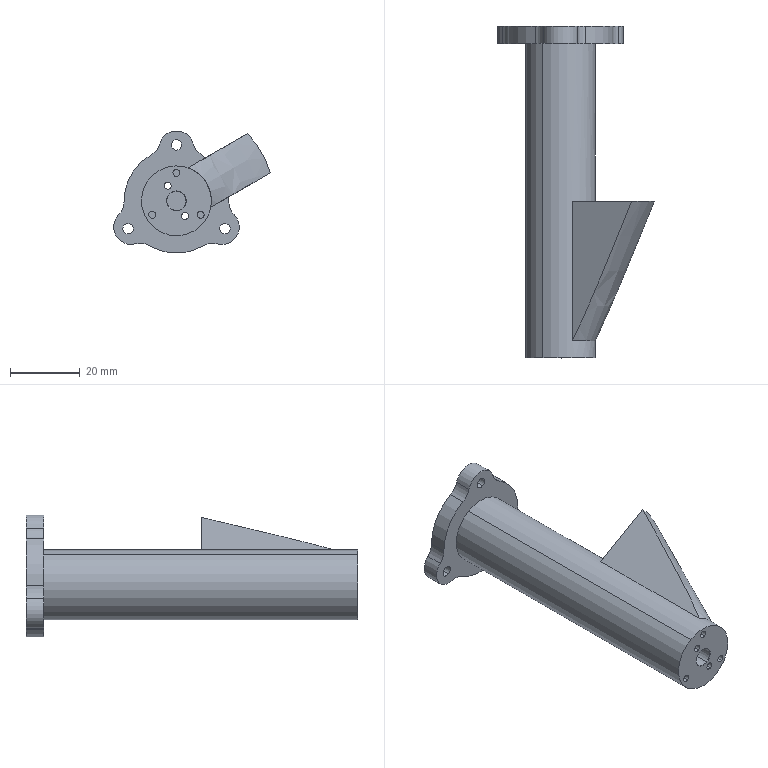Component | SolidWorks | Nozzle1-1 | 1 solid | 58 faces | box 44.86 x 95 x 35 mm | volume 30330 mm3 | cylinder 41 | plane 12 | cone 5 | commonest cylinder face diameters 10 x11 2 x10 3 x8 30 x4 5 x2 13 x2 20 x2 5.5 x2
build123d program:
from build123d import *

# Parameters (mm, degrees)
CUT_EXTRUDE1_REACH       = 101.121
SKETCH4_R                = 1
CUT_EXTRUDE3_START       = -5
SKETCH5_R                = 20
CUT_EXTRUDE3_DEPTH       = 5
FILLET1_R                = 5
SKETCH6_R                = 2.75
CUT_EXTRUDE4_DEPTH       = 20
CUT_EXTRUDE5_REACH       = 100.735
SKETCH7_R                = 1.5
SKETCH12_R               = 1
CUT_EXTRUDE8_DEPTH       = 5
CHAMFER2_SIZE            = 0.08
BOSS_EXTRUDE1_REACH      = 74.782
BOSS_EXTRUDE1_END_RADIUS = 10
SKETCH16_W               = 40
SKETCH16_H               = 13
CUT_EXTRUDE7_REACH       = 77.197
CUT_EXTRUDE7_END_RADIUS  = 2.75
SKETCH11_R               = 1.5
SKETCH25_R               = 2.5
CUT_EXTRUDE10_DEPTH      = 20


with BuildPart() as part:
    # Sketch2 → Revolve1 (revolve)
    with BuildSketch(Plane.XY, mode=Mode.PRIVATE) as revolve1_sk:
        Polygon((-49.735, 0), (45.265, 0), (45.265, 10), (-44.735, 10), (-44.735, 20), (-49.735, 20), align=None)
    revolve(revolve1_sk.sketch.rotate(Axis((-49.735, 0, 0), (1, 0, 0)), 90), axis=Axis((-49.735, 0, 0), (1, 0, 0)))

    # Sketch3 → Cut-Revolve1 (revolve, cut)
    with BuildSketch(Plane(origin=(0, 0, 0), x_dir=(1, 0, 0), z_dir=(0, 1, 0)), mode=Mode.PRIVATE) as cut_revolve1_sk:
        Polygon((-44.735, 6.5), (-49.735, 10), (-49.735, 0), (-9.735, 0), (-9.735, 6.5), align=None)
    revolve(cut_revolve1_sk.sketch.rotate(Axis((-53.807, 0, 0), (1, 0, 0)), 180), axis=Axis((-53.807, 0, 0), (1, 0, 0)), mode=Mode.SUBTRACT)

    # Sketch4 → Cut-Extrude1 (cut, up to next)
    with BuildSketch(Plane(origin=(45.265, 0, 0), x_dir=(0, 0, -1), z_dir=(1, 0, 0)), mode=Mode.PRIVATE) as cut_extrude1_sk1:
        with Locations((5, 0)):
            Circle(SKETCH4_R)
    cut_extrude1_tool1 = extrude(cut_extrude1_sk1.sketch, amount=-CUT_EXTRUDE1_REACH, mode=Mode.PRIVATE) & part.part
    # Sketch4 → Cut-Extrude1 (cut, up to next)
    with BuildSketch(Plane(origin=(45.265, 0, 0), x_dir=(0, 0, -1), z_dir=(1, 0, 0)), mode=Mode.PRIVATE) as cut_extrude1_sk2:
        with Locations(Location((-5, 0, 0), (0, 0, 180))):
            Circle(SKETCH4_R)
    cut_extrude1_tool2 = extrude(cut_extrude1_sk2.sketch, amount=-CUT_EXTRUDE1_REACH, mode=Mode.PRIVATE) & part.part
    add(cut_extrude1_tool1.solids().sort_by_distance((45.265, 0, -5))[0], mode=Mode.SUBTRACT)
    add(cut_extrude1_tool2.solids().sort_by_distance((45.265, 0, 5))[0], mode=Mode.SUBTRACT)

    # Sketch5 → Cut-Extrude3 (cut)
    with BuildSketch(Plane.ZY.offset(49.735).offset(CUT_EXTRUDE3_START)):
        Circle(SKETCH5_R)
        with BuildLine():
            ThreePointArc((4.93, 14.167), (0, 20), (-4.93, 14.167))
            ThreePointArc((-4.93, 14.167), (-12.99, 7.5), (-14.734, -2.814))
            ThreePointArc((-14.734, -2.814), (-17.321, -10), (-9.804, -11.353))
            ThreePointArc((-9.804, -11.353), (0, -15), (9.804, -11.353))
            ThreePointArc((9.804, -11.353), (17.321, -10), (14.734, -2.814))
            ThreePointArc((14.734, -2.814), (12.99, 7.5), (4.93, 14.167))
        make_face(mode=Mode.SUBTRACT)
    extrude(amount=CUT_EXTRUDE3_DEPTH, mode=Mode.SUBTRACT)

    # Fillet1
    fillet1_edges = [part.edges().sort_by_distance(p)[0] for p in [
        (-47.235, 14.167, -4.93),
        (-47.235, -2.814, -14.734),
        (-47.235, -2.814, 14.734),
        (-47.235, 14.167, 4.93),
        (-47.235, -11.353, -9.804),
        (-47.235, -11.353, 9.804),
    ]]
    fillet(fillet1_edges, radius=FILLET1_R)

    # Sketch6 → Cut-Extrude4 (cut)
    with BuildSketch(Plane(origin=(45.265, 0, 0), x_dir=(0, 0, -1), z_dir=(1, 0, 0))):
        Circle(SKETCH6_R)
    extrude(amount=-CUT_EXTRUDE4_DEPTH, mode=Mode.SUBTRACT)

    # Sketch7 → Cut-Extrude5 (cut, up to next)
    with BuildSketch(Plane.ZY.offset(49.735), mode=Mode.PRIVATE) as cut_extrude5_sk1:
        with Locations((0, 16)):
            Circle(SKETCH7_R)
    cut_extrude5_tool1 = extrude(cut_extrude5_sk1.sketch, amount=-CUT_EXTRUDE5_REACH, mode=Mode.PRIVATE) & part.part
    # Sketch7 → Cut-Extrude5 (cut, up to next)
    with BuildSketch(Plane.ZY.offset(49.735), mode=Mode.PRIVATE) as cut_extrude5_sk2:
        with Locations((13.856, -8)):
            Circle(SKETCH7_R)
    cut_extrude5_tool2 = extrude(cut_extrude5_sk2.sketch, amount=-CUT_EXTRUDE5_REACH, mode=Mode.PRIVATE) & part.part
    # Sketch7 → Cut-Extrude5 (cut, up to next)
    with BuildSketch(Plane.ZY.offset(49.735), mode=Mode.PRIVATE) as cut_extrude5_sk3:
        with Locations((-13.856, -8)):
            Circle(SKETCH7_R)
    cut_extrude5_tool3 = extrude(cut_extrude5_sk3.sketch, amount=-CUT_EXTRUDE5_REACH, mode=Mode.PRIVATE) & part.part
    add(cut_extrude5_tool1.solids().sort_by_distance((-49.735, 16, 0))[0], mode=Mode.SUBTRACT)
    add(cut_extrude5_tool2.solids().sort_by_distance((-49.735, -8, 13.856))[0], mode=Mode.SUBTRACT)
    add(cut_extrude5_tool3.solids().sort_by_distance((-49.735, -8, -13.856))[0], mode=Mode.SUBTRACT)

    # Sketch12 → Cut-Extrude8 (cut)
    with BuildSketch(Plane(origin=(45.265, 0, 0), x_dir=(0, 0, -1), z_dir=(1, 0, 0))):
        with Locations((0, 8)):
            Circle(SKETCH12_R)
        with Locations((6.928, -4)):
            Circle(SKETCH12_R)
        with Locations((-6.928, -4)):
            Circle(SKETCH12_R)
    extrude(amount=-CUT_EXTRUDE8_DEPTH, mode=Mode.SUBTRACT)

    # Chamfer2
    chamfer2_edges = [part.edges().sort_by_distance(p)[0] for p in [
        (45.265, 0, 2.75),
    ]]
    chamfer(chamfer2_edges, length=CHAMFER2_SIZE)

    # Boss-Extrude1: up to this cylinder (the profile starts outside it)
    boss_extrude1_end = Plane(origin=(20.382, 0, 0), z_dir=(-1, 0, 0)) * Cylinder(BOSS_EXTRUDE1_END_RADIUS, 170.564, mode=Mode.PRIVATE)
    # Sketch16 → Boss-Extrude1 (add, up to the surface)
    with BuildSketch(Plane(origin=(0, -30, 0), x_dir=(1, 0, 0), z_dir=(0, 1, 0)), mode=Mode.PRIVATE) as boss_extrude1_sk1:
        with Locations((20.382, 0)):
            Rectangle(SKETCH16_W, SKETCH16_H)
    boss_extrude1_tool1 = extrude(boss_extrude1_sk1.sketch, amount=BOSS_EXTRUDE1_REACH, mode=Mode.PRIVATE) - boss_extrude1_end
    add(boss_extrude1_tool1.solids().sort_by_distance((20.382, -30, 0))[0])

    # Sketch18 → Cut-Revolve4 (revolve, cut)
    with BuildSketch(Plane.XY, mode=Mode.PRIVATE) as cut_revolve4_sk:
        Polygon((40.382, -10), (-9.791, -32.631), (40.382, -32.631), align=None)
    revolve(cut_revolve4_sk.sketch.rotate(Axis((-28.557, 0, 0), (1, 0, 0)), 270), axis=Axis((-28.557, 0, 0), (1, 0, 0)), mode=Mode.SUBTRACT)

    # Cut-Extrude7: up to this cylinder (the profile starts outside it)
    cut_extrude7_end = Plane(origin=(-15.153, 0, 0), z_dir=(1, 0, 0)) * Cylinder(CUT_EXTRUDE7_END_RADIUS, 160.894, mode=Mode.PRIVATE)
    # Sketch11 → Cut-Extrude7 (cut, up to the surface)
    with BuildSketch(Plane(origin=(-15.158, -20.987, 0), x_dir=(0, 0, -1), z_dir=(0.9397, 0.342, 0)), mode=Mode.PRIVATE) as cut_extrude7_sk1:
        with Locations(Location((0, -0.01473, 0), (0, 0, 270))):
            Circle(SKETCH11_R)
    cut_extrude7_tool1 = extrude(cut_extrude7_sk1.sketch, amount=CUT_EXTRUDE7_REACH, mode=Mode.PRIVATE) - cut_extrude7_end
    add(cut_extrude7_tool1.solids().sort_by_distance((-15.153, -21.001, 0))[0], mode=Mode.SUBTRACT)

    # Sketch25 → Cut-Extrude10 (cut)
    with BuildSketch(Plane(origin=(-15.158, -20.987, 0), x_dir=(0, 0, -1), z_dir=(0.9397, 0.342, 0))):
        with Locations(Location((0, -0.01473, 0), (0, 0, 270))):
            Circle(SKETCH25_R)
    extrude(amount=CUT_EXTRUDE10_DEPTH, mode=Mode.SUBTRACT)


solid = part.part

# Placed as in the assembly
solid = solid.moved(Location((-5.981, -61.229, 160), (-180, 30, 90)))